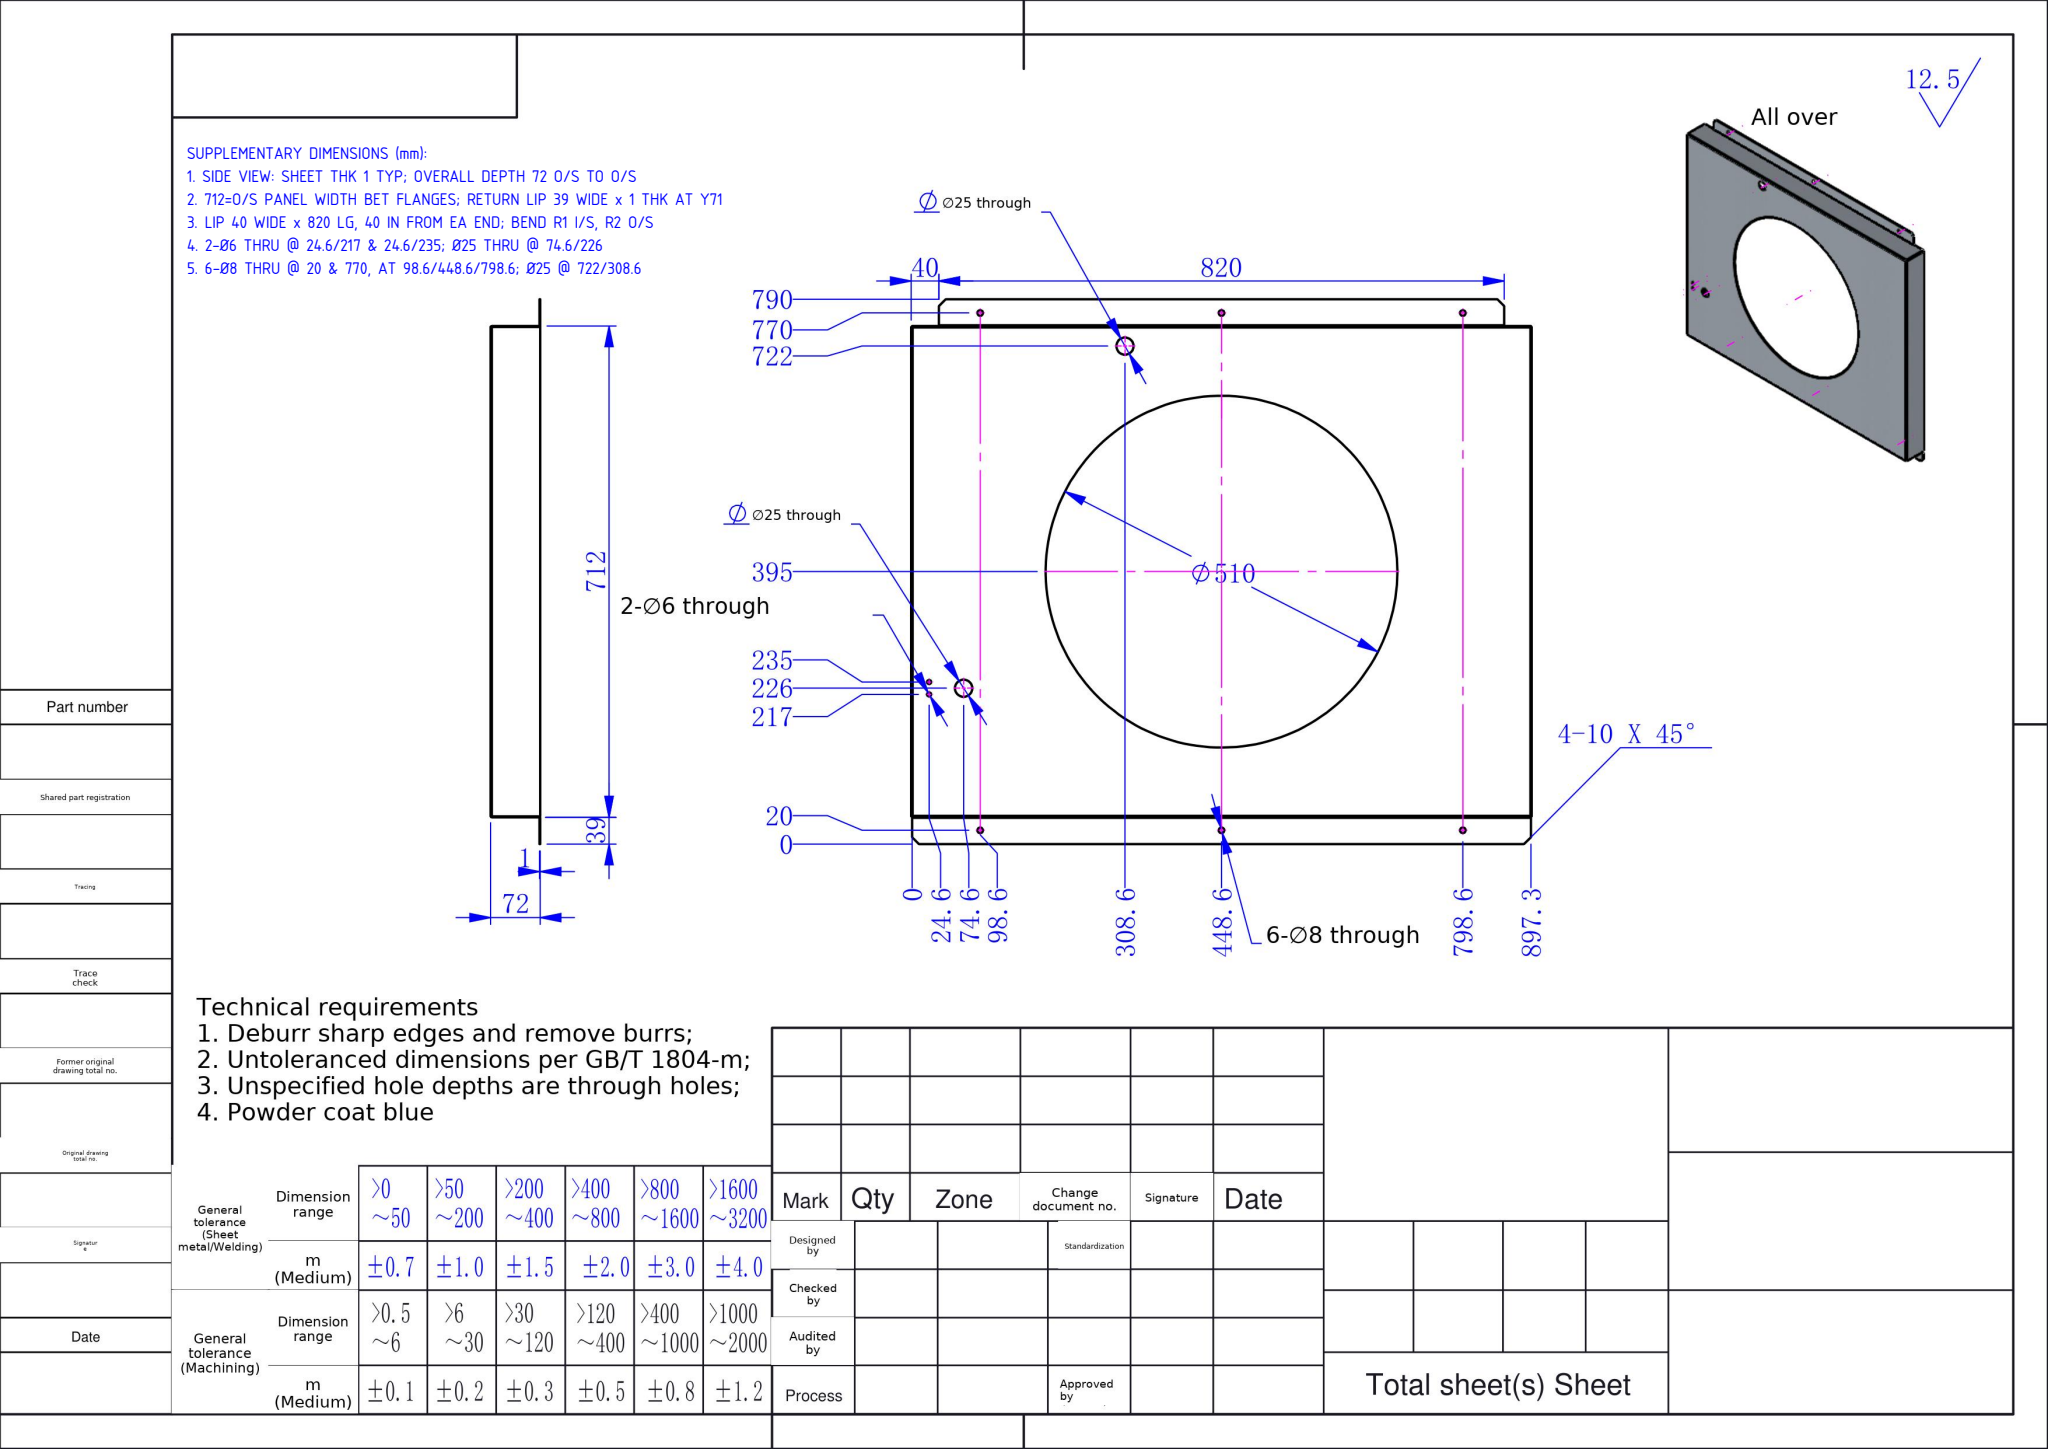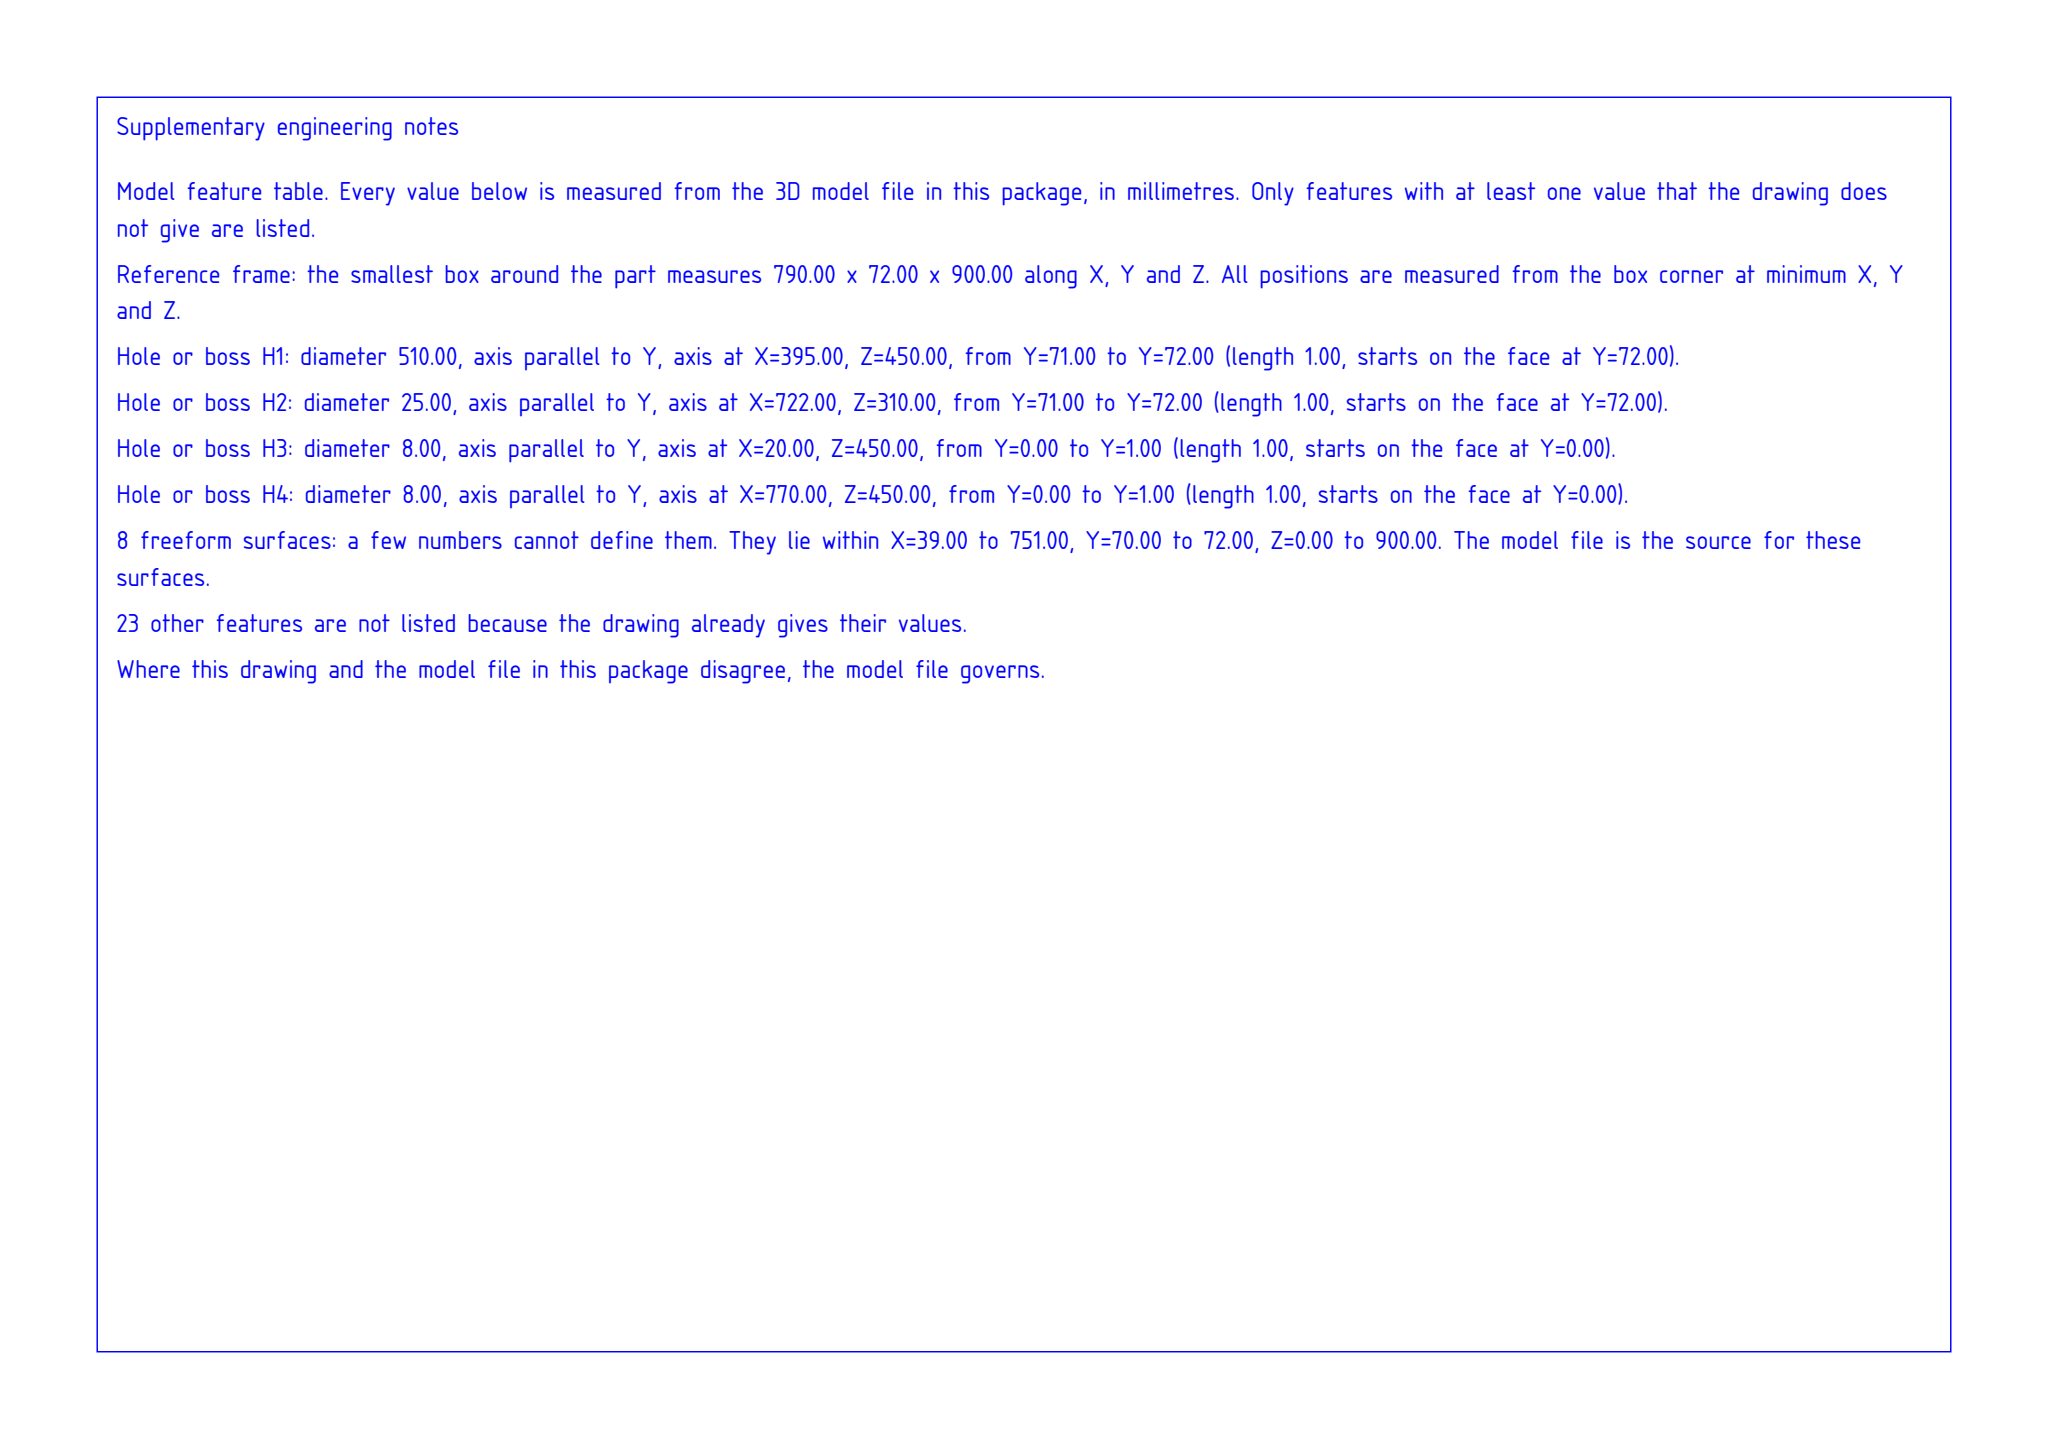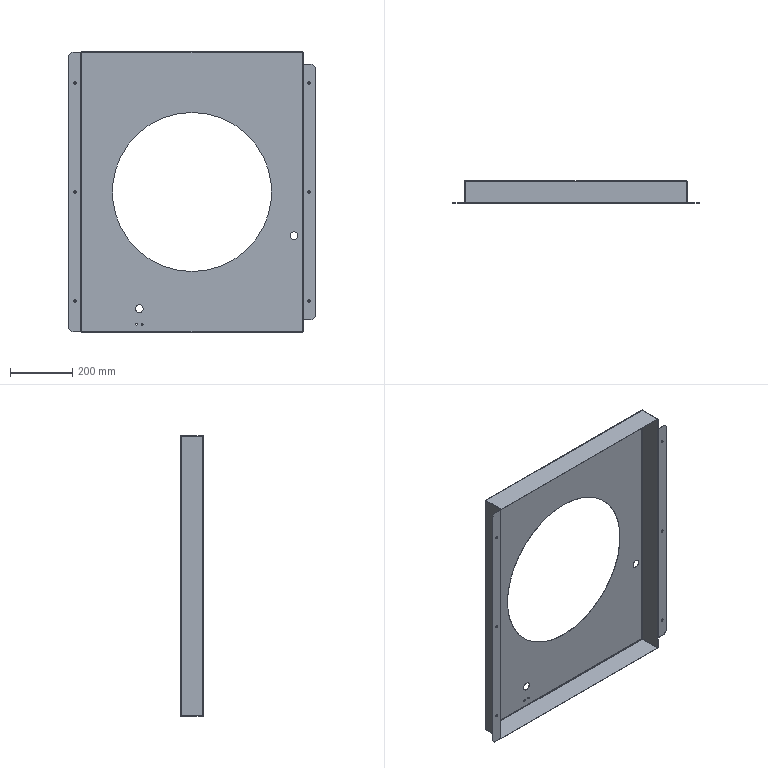Part | SolidWorks | mm | 1 solid | 88 faces | box 790 x 72 x 900 mm | volume 726899 mm3 | plane 46 | cylinder 34 | spline 8 | commonest cylinder face diameters 8 x12 4 x6 2 x6 25 x4 6 x4 510 x2